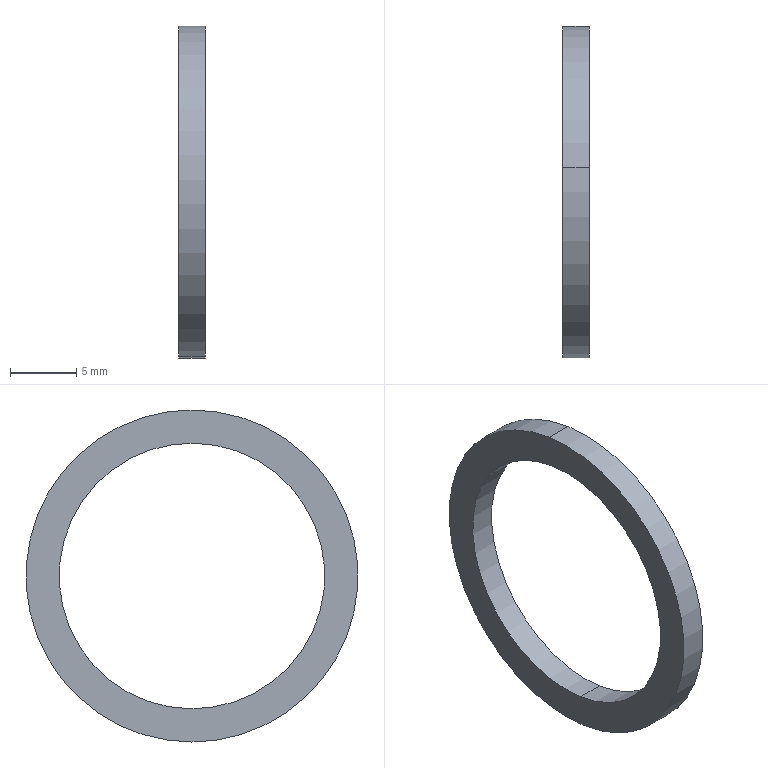Component | SolidWorks | Washer12-1 | 1 solid | 6 faces | box 2 x 25 x 25 mm | volume 353 mm3 | cylinder 4 | plane 2 | commonest cylinder face diameters 20 x2 25 x2
build123d program:
from build123d import *

# Parameters (mm, degrees)
SKETCH1_R           = 12.5
SKETCH1_R_2         = 10
BOSS_EXTRUDE1_DEPTH = 2


with BuildPart() as part:
    # Sketch1 → Boss-Extrude1 (new body)
    with BuildSketch(Plane.XY):
        with Locations((15, 150)):
            Circle(SKETCH1_R)
        with Locations((15, 150)):
            Circle(SKETCH1_R_2, mode=Mode.SUBTRACT)
    extrude(amount=BOSS_EXTRUDE1_DEPTH)


solid = part.part

# Placed as in the assembly
solid = solid.moved(Location((149.052, 0, 0), (0, 90, 0)))
STEP:
#1=CARTESIAN_POINT('',(5.947,5.964,-0.2012));
#2=VERTEX_POINT('',#1);
#3=CARTESIAN_POINT('',(5.947,5.847,-0.9799));
#4=VERTEX_POINT('',#3);
#5=CARTESIAN_POINT('',(5.947,5.906,-0.5906));
#6=DIRECTION('',(1.,0.,0.));
#7=DIRECTION('',(0.,-0.1487,-0.9889));
#8=AXIS2_PLACEMENT_3D('',#5,#6,#7);
#9=CIRCLE('',#8,0.3937);
#10=EDGE_CURVE('',#2,#4,#9,.T.);
#11=ORIENTED_EDGE('',*,*,#10,.T.);
#12=CARTESIAN_POINT('',(5.868,5.847,-0.9799));
#13=VERTEX_POINT('',#12);
#14=CARTESIAN_POINT('',(5.947,5.847,-0.9799));
#15=DIRECTION('',(-1.,0.,0.));
#16=VECTOR('',#15,39.37);
#17=LINE('',#14,#16);
#18=EDGE_CURVE('',#4,#13,#17,.T.);
#19=ORIENTED_EDGE('',*,*,#18,.T.);
#20=CARTESIAN_POINT('',(5.868,5.964,-0.2012));
#21=VERTEX_POINT('',#20);
#22=CARTESIAN_POINT('',(5.868,5.906,-0.5906));
#23=DIRECTION('',(1.,0.,0.));
#24=DIRECTION('',(0.,-0.1487,-0.9889));
#25=AXIS2_PLACEMENT_3D('',#22,#23,#24);
#26=CIRCLE('',#25,0.3937);
#27=EDGE_CURVE('',#21,#13,#26,.T.);
#28=ORIENTED_EDGE('',*,*,#27,.F.);
#29=CARTESIAN_POINT('',(5.947,5.964,-0.2012));
#30=DIRECTION('',(-1.,0.,0.));
#31=VECTOR('',#30,39.37);
#32=LINE('',#29,#31);
#33=EDGE_CURVE('',#2,#21,#32,.T.);
#34=ORIENTED_EDGE('',*,*,#33,.F.);
#35=EDGE_LOOP('',(#11,#19,#28,#34));
#36=FACE_OUTER_BOUND('',#35,.T.);
#37=CARTESIAN_POINT('',(5.947,5.906,-0.5906));
#38=DIRECTION('',(-1.,0.,0.));
#39=DIRECTION('',(0.,0.1487,0.9889));
#40=AXIS2_PLACEMENT_3D('',#37,#38,#39);
#41=CYLINDRICAL_SURFACE('',#40,0.3937);
#42=ADVANCED_FACE('',(#36),#41,.F.);
#43=CARTESIAN_POINT('',(5.947,5.832,-1.077));
#44=VERTEX_POINT('',#43);
#45=CARTESIAN_POINT('',(5.947,5.979,-0.1039));
#46=VERTEX_POINT('',#45);
#47=CARTESIAN_POINT('',(5.947,5.906,-0.5906));
#48=DIRECTION('',(1.,0.,0.));
#49=DIRECTION('',(0.,-0.1487,-0.9889));
#50=AXIS2_PLACEMENT_3D('',#47,#48,#49);
#51=CIRCLE('',#50,0.4921);
#52=EDGE_CURVE('',#44,#46,#51,.T.);
#53=ORIENTED_EDGE('',*,*,#52,.F.);
#54=CARTESIAN_POINT('',(5.868,5.832,-1.077));
#55=VERTEX_POINT('',#54);
#56=CARTESIAN_POINT('',(5.947,5.832,-1.077));
#57=DIRECTION('',(-1.,0.,0.));
#58=VECTOR('',#57,39.37);
#59=LINE('',#56,#58);
#60=EDGE_CURVE('',#44,#55,#59,.T.);
#61=ORIENTED_EDGE('',*,*,#60,.T.);
#62=CARTESIAN_POINT('',(5.868,5.979,-0.1039));
#63=VERTEX_POINT('',#62);
#64=CARTESIAN_POINT('',(5.868,5.906,-0.5906));
#65=DIRECTION('',(1.,0.,0.));
#66=DIRECTION('',(0.,-0.1487,-0.9889));
#67=AXIS2_PLACEMENT_3D('',#64,#65,#66);
#68=CIRCLE('',#67,0.4921);
#69=EDGE_CURVE('',#55,#63,#68,.T.);
#70=ORIENTED_EDGE('',*,*,#69,.T.);
#71=CARTESIAN_POINT('',(5.947,5.979,-0.1039));
#72=DIRECTION('',(-1.,0.,0.));
#73=VECTOR('',#72,39.37);
#74=LINE('',#71,#73);
#75=EDGE_CURVE('',#46,#63,#74,.T.);
#76=ORIENTED_EDGE('',*,*,#75,.F.);
#77=EDGE_LOOP('',(#53,#61,#70,#76));
#78=FACE_OUTER_BOUND('',#77,.T.);
#79=CARTESIAN_POINT('',(5.947,5.906,-0.5906));
#80=DIRECTION('',(-1.,0.,0.));
#81=DIRECTION('',(0.,0.1487,0.9889));
#82=AXIS2_PLACEMENT_3D('',#79,#80,#81);
#83=CYLINDRICAL_SURFACE('',#82,0.4921);
#84=ADVANCED_FACE('',(#78),#83,.T.);
#85=CARTESIAN_POINT('',(5.947,5.906,-0.5906));
#86=DIRECTION('',(1.,0.,0.));
#87=DIRECTION('',(0.,-0.1487,-0.9889));
#88=AXIS2_PLACEMENT_3D('',#85,#86,#87);
#89=CIRCLE('',#88,0.4921);
#90=EDGE_CURVE('',#46,#44,#89,.T.);
#91=ORIENTED_EDGE('',*,*,#90,.T.);
#92=ORIENTED_EDGE('',*,*,#52,.T.);
#93=EDGE_LOOP('',(#91,#92));
#94=FACE_OUTER_BOUND('',#93,.T.);
#95=ORIENTED_EDGE('',*,*,#10,.F.);
#96=CARTESIAN_POINT('',(5.947,5.906,-0.5906));
#97=DIRECTION('',(1.,0.,0.));
#98=DIRECTION('',(0.,-0.1487,-0.9889));
#99=AXIS2_PLACEMENT_3D('',#96,#97,#98);
#100=CIRCLE('',#99,0.3937);
#101=EDGE_CURVE('',#4,#2,#100,.T.);
#102=ORIENTED_EDGE('',*,*,#101,.F.);
#103=EDGE_LOOP('',(#95,#102));
#104=FACE_BOUND('',#103,.T.);
#105=CARTESIAN_POINT('',(5.947,5.906,-0.5906));
#106=DIRECTION('',(1.,0.,0.));
#107=DIRECTION('',(0.,-0.1487,-0.9889));
#108=AXIS2_PLACEMENT_3D('',#105,#106,#107);
#109=PLANE('',#108);
#110=ADVANCED_FACE('',(#94,#104),#109,.T.);
#111=CARTESIAN_POINT('',(5.868,5.906,-0.5906));
#112=DIRECTION('',(1.,0.,0.));
#113=DIRECTION('',(0.,-0.1487,-0.9889));
#114=AXIS2_PLACEMENT_3D('',#111,#112,#113);
#115=CIRCLE('',#114,0.4921);
#116=EDGE_CURVE('',#63,#55,#115,.T.);
#117=ORIENTED_EDGE('',*,*,#116,.F.);
#118=ORIENTED_EDGE('',*,*,#69,.F.);
#119=EDGE_LOOP('',(#117,#118));
#120=FACE_OUTER_BOUND('',#119,.T.);
#121=ORIENTED_EDGE('',*,*,#27,.T.);
#122=CARTESIAN_POINT('',(5.868,5.906,-0.5906));
#123=DIRECTION('',(1.,0.,0.));
#124=DIRECTION('',(0.,-0.1487,-0.9889));
#125=AXIS2_PLACEMENT_3D('',#122,#123,#124);
#126=CIRCLE('',#125,0.3937);
#127=EDGE_CURVE('',#13,#21,#126,.T.);
#128=ORIENTED_EDGE('',*,*,#127,.T.);
#129=EDGE_LOOP('',(#121,#128));
#130=FACE_BOUND('',#129,.T.);
#131=CARTESIAN_POINT('',(5.868,5.906,-0.5906));
#132=DIRECTION('',(1.,0.,0.));
#133=DIRECTION('',(0.,-0.1487,-0.9889));
#134=AXIS2_PLACEMENT_3D('',#131,#132,#133);
#135=PLANE('',#134);
#136=ADVANCED_FACE('',(#120,#130),#135,.F.);
#137=ORIENTED_EDGE('',*,*,#60,.F.);
#138=ORIENTED_EDGE('',*,*,#90,.F.);
#139=ORIENTED_EDGE('',*,*,#75,.T.);
#140=ORIENTED_EDGE('',*,*,#116,.T.);
#141=EDGE_LOOP('',(#137,#138,#139,#140));
#142=FACE_OUTER_BOUND('',#141,.T.);
#143=CARTESIAN_POINT('',(5.947,5.906,-0.5906));
#144=DIRECTION('',(-1.,0.,0.));
#145=DIRECTION('',(0.,0.1487,0.9889));
#146=AXIS2_PLACEMENT_3D('',#143,#144,#145);
#147=CYLINDRICAL_SURFACE('',#146,0.4921);
#148=ADVANCED_FACE('',(#142),#147,.T.);
#149=ORIENTED_EDGE('',*,*,#18,.F.);
#150=ORIENTED_EDGE('',*,*,#101,.T.);
#151=ORIENTED_EDGE('',*,*,#33,.T.);
#152=ORIENTED_EDGE('',*,*,#127,.F.);
#153=EDGE_LOOP('',(#149,#150,#151,#152));
#154=FACE_OUTER_BOUND('',#153,.T.);
#155=CARTESIAN_POINT('',(5.947,5.906,-0.5906));
#156=DIRECTION('',(-1.,0.,0.));
#157=DIRECTION('',(0.,0.1487,0.9889));
#158=AXIS2_PLACEMENT_3D('',#155,#156,#157);
#159=CYLINDRICAL_SURFACE('',#158,0.3937);
#160=ADVANCED_FACE('',(#154),#159,.F.);
#161=CLOSED_SHELL('',(#42,#84,#110,#136,#148,#160));
#162=MANIFOLD_SOLID_BREP('',#161);
#163=CARTESIAN_POINT('',(0.,0.,0.));
#164=DIRECTION('',(0.,0.,1.));
#165=DIRECTION('',(1.,0.,0.));
#166=AXIS2_PLACEMENT_3D('',#163,#164,#165);
#167=(LENGTH_UNIT()NAMED_UNIT(*)SI_UNIT($,.METRE.));
#168=LENGTH_MEASURE_WITH_UNIT(LENGTH_MEASURE(0.0254),#167);
#169=DIMENSIONAL_EXPONENTS(1.,0.,0.,0.,0.,0.,0.);
#170=(CONVERSION_BASED_UNIT('',#168)LENGTH_UNIT()NAMED_UNIT(#169));
#171=UNCERTAINTY_MEASURE_WITH_UNIT(LENGTH_MEASURE(0.00001),#170,'','');
#172=(NAMED_UNIT(*)PLANE_ANGLE_UNIT()SI_UNIT($,.RADIAN.));
#173=(NAMED_UNIT(*)SI_UNIT($,.STERADIAN.)SOLID_ANGLE_UNIT());
#174=(GEOMETRIC_REPRESENTATION_CONTEXT(3)GLOBAL_UNCERTAINTY_ASSIGNED_CONTEXT((#171))GLOBAL_UNIT_ASSIGNED_CONTEXT((#170,#172,#173))REPRESENTATION_CONTEXT('',''));
#175=ADVANCED_BREP_SHAPE_REPRESENTATION('',(#162,#166),#174);
#176=COLOUR_RGB('',0.7922,0.8196,0.9333);
#177=FILL_AREA_STYLE_COLOUR('',#176);
#178=FILL_AREA_STYLE('',(#177));
#179=SURFACE_STYLE_FILL_AREA(#178);
#180=SURFACE_SIDE_STYLE('',(#179));
#181=SURFACE_STYLE_USAGE(.BOTH.,#180);
#182=PRESENTATION_STYLE_ASSIGNMENT((#181));
#183=STYLED_ITEM('',(#182),#162);
#184=PRESENTATION_LAYER_ASSIGNMENT('','',(#183));
#185=(LENGTH_UNIT()NAMED_UNIT(*)SI_UNIT($,.METRE.));
#186=LENGTH_MEASURE_WITH_UNIT(LENGTH_MEASURE(0.0254),#185);
#187=DIMENSIONAL_EXPONENTS(1.,0.,0.,0.,0.,0.,0.);
#188=(CONVERSION_BASED_UNIT('',#186)LENGTH_UNIT()NAMED_UNIT(#187));
#189=UNCERTAINTY_MEASURE_WITH_UNIT(LENGTH_MEASURE(0.00001),#188,'','');
#190=(NAMED_UNIT(*)PLANE_ANGLE_UNIT()SI_UNIT($,.RADIAN.));
#191=(NAMED_UNIT(*)SI_UNIT($,.STERADIAN.)SOLID_ANGLE_UNIT());
#192=(GEOMETRIC_REPRESENTATION_CONTEXT(3)GLOBAL_UNCERTAINTY_ASSIGNED_CONTEXT((#189))GLOBAL_UNIT_ASSIGNED_CONTEXT((#188,#190,#191))REPRESENTATION_CONTEXT('',''));
#193=MECHANICAL_DESIGN_GEOMETRIC_PRESENTATION_REPRESENTATION('',(#183),#192);